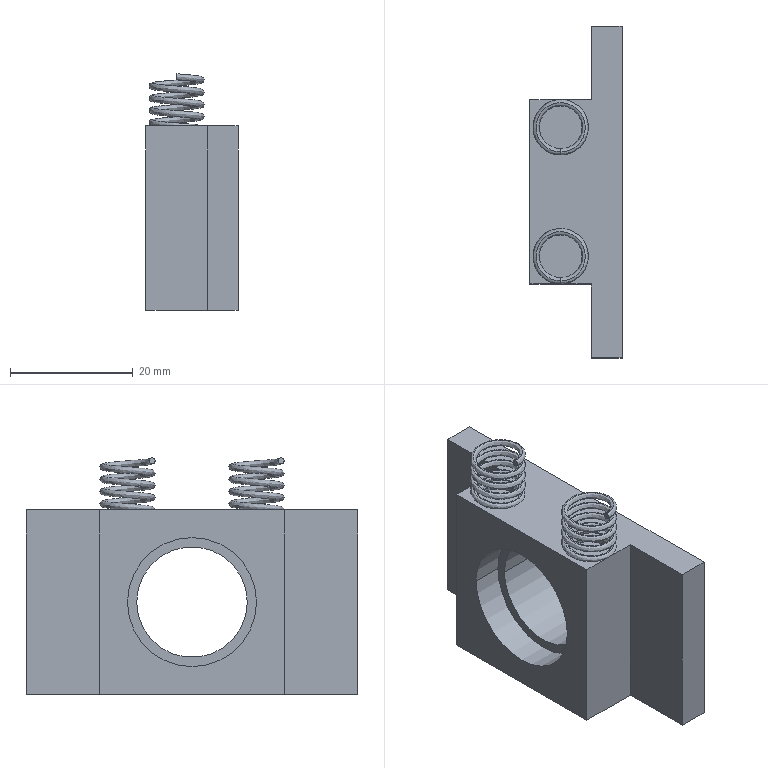Component | SolidWorks | SupportPlate1-1 | 1 solid | 31 faces | volume 12799 mm3 | plane 17 | cylinder 10 | spline 4 | commonest cylinder face diameters 8 x6 18 x2 21 x2